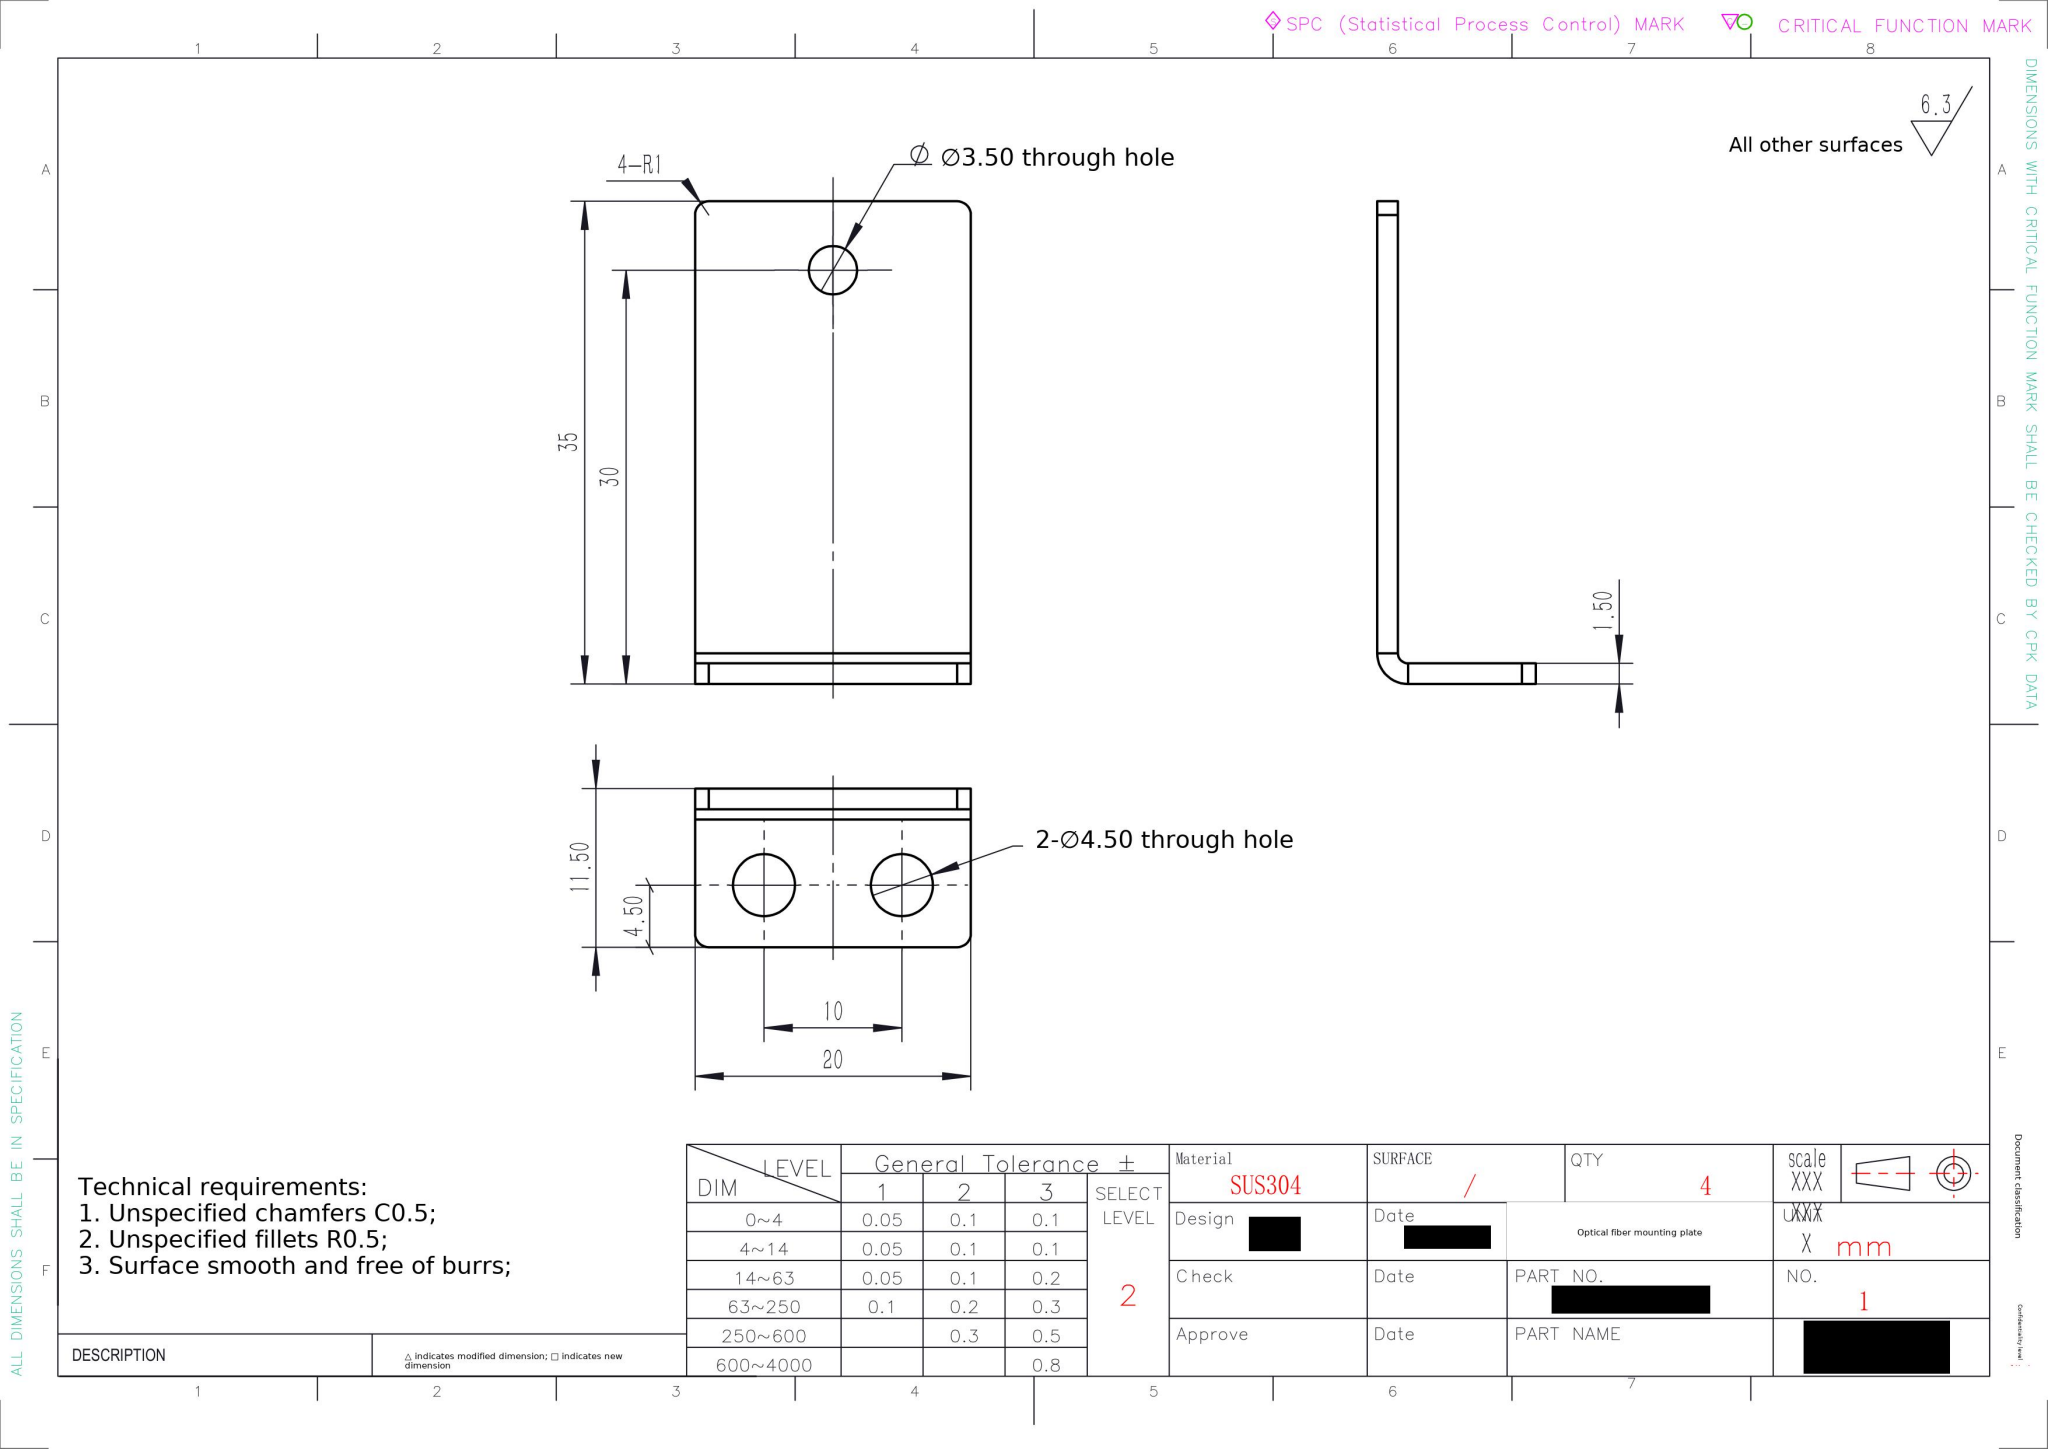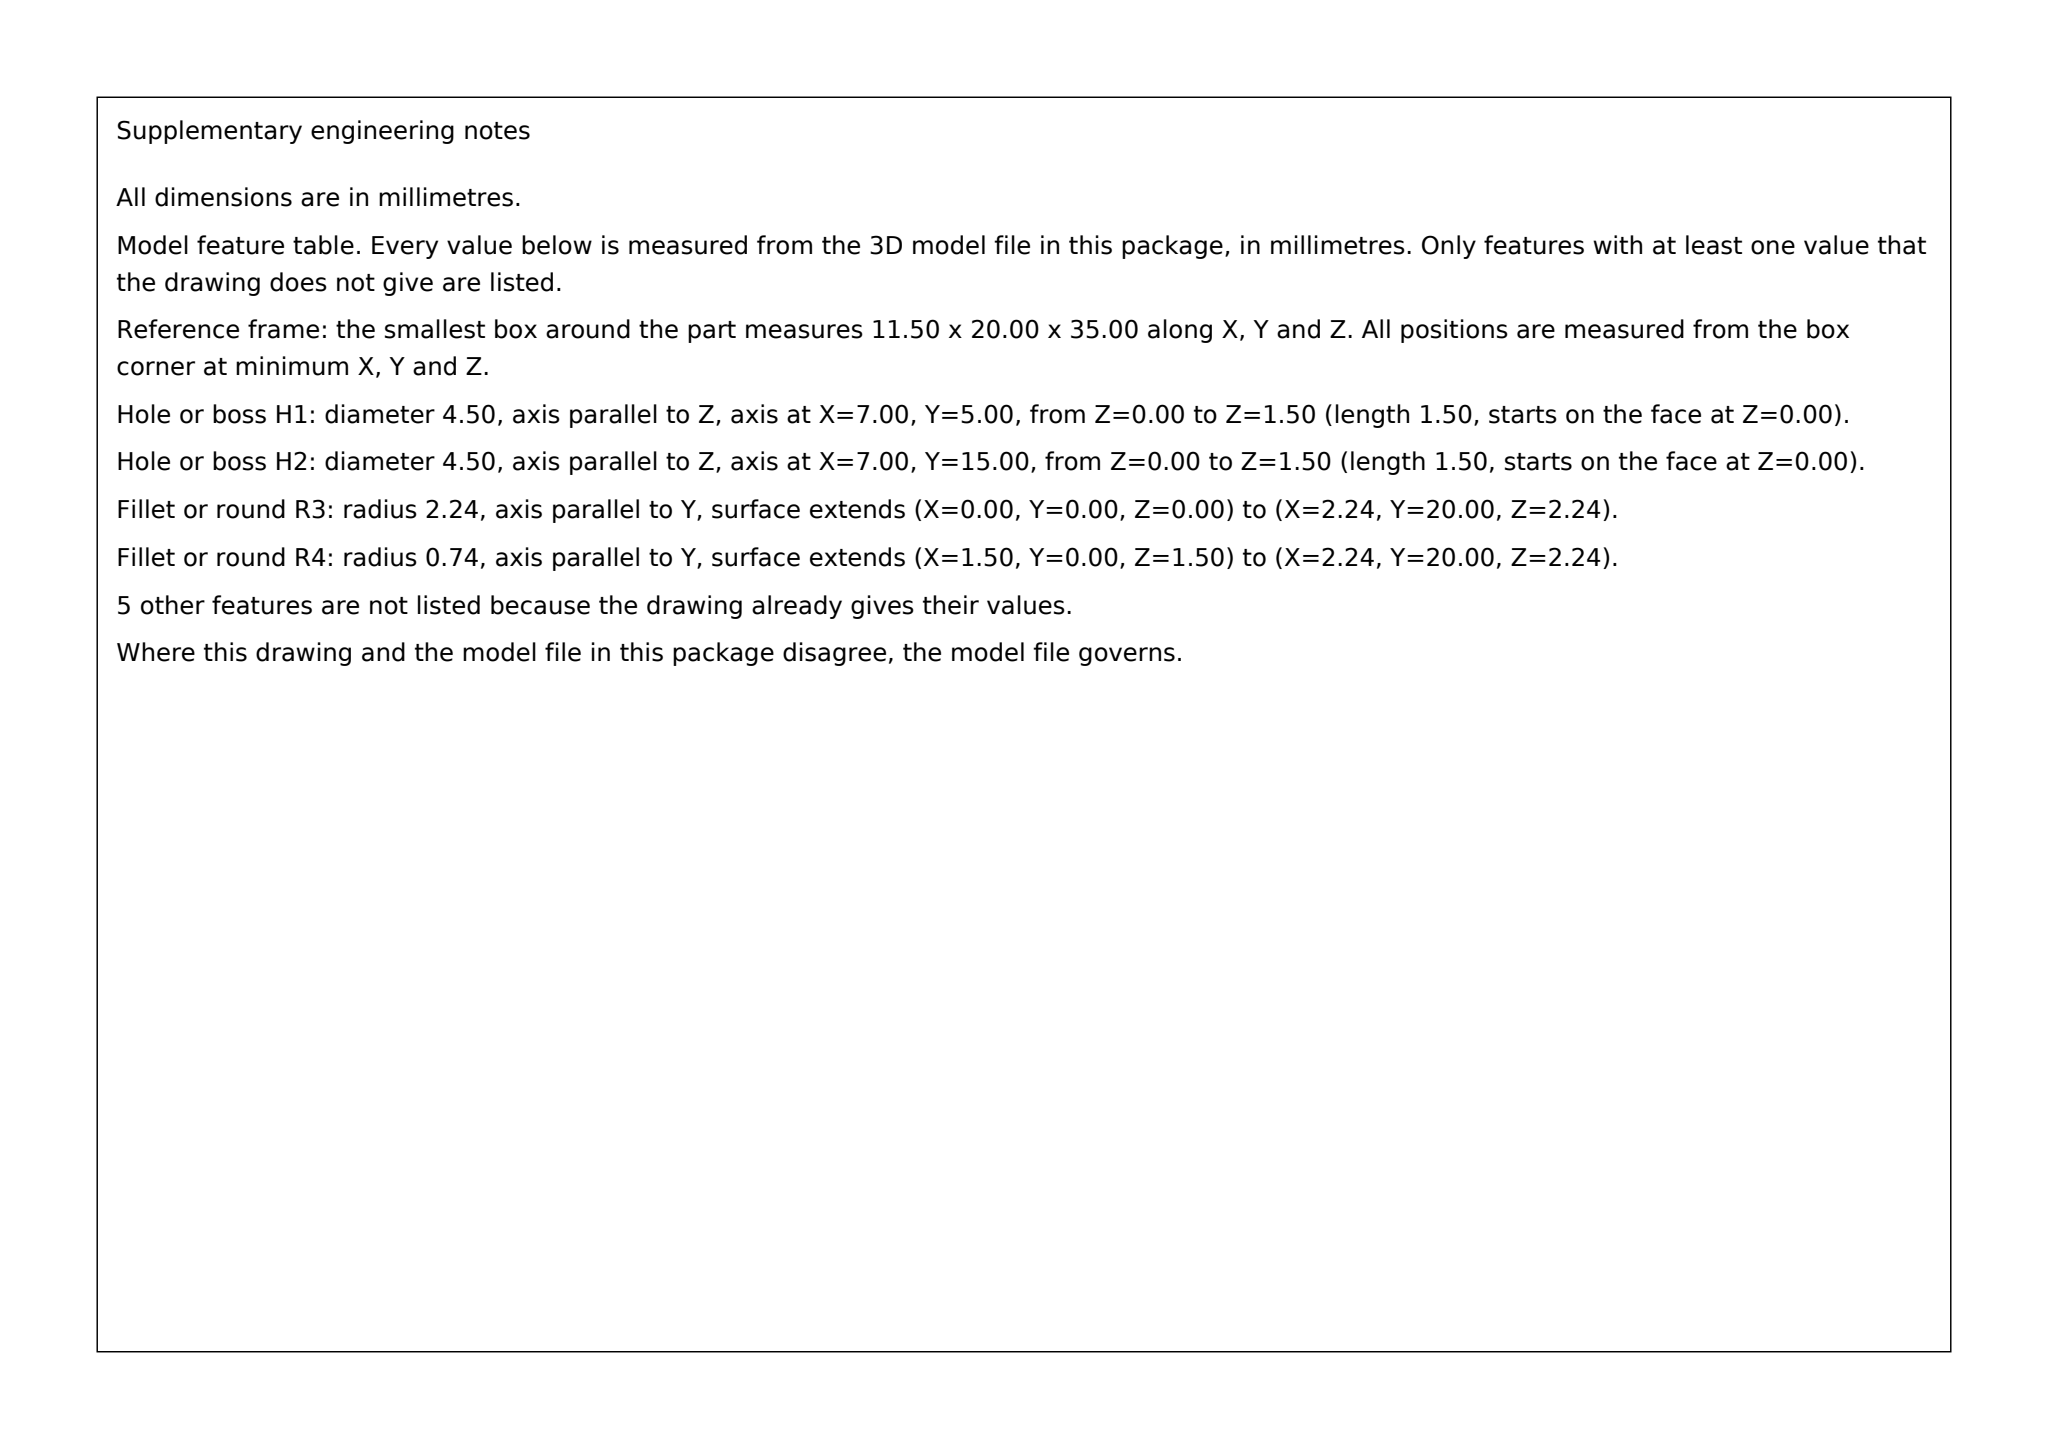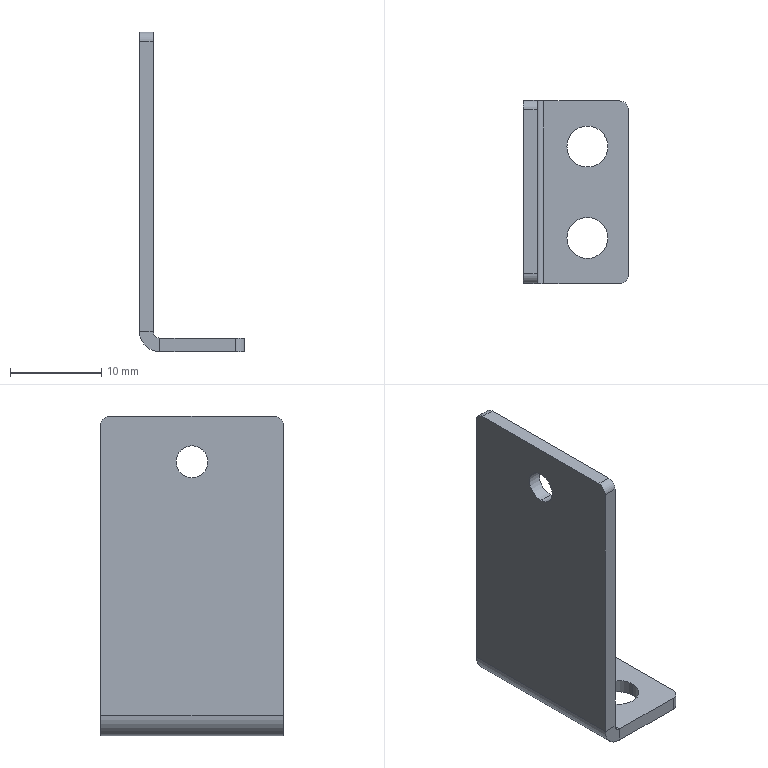Part | SolidWorks | mm | material SUS304 | 1 solid | 24 faces | box 11.5 x 20 x 35 mm | volume 1267 mm3 | cylinder 12 | plane 12 | commonest cylinder face diameters 4.5 x4 2 x4 3.5 x2 4.473 x1 1.473 x1